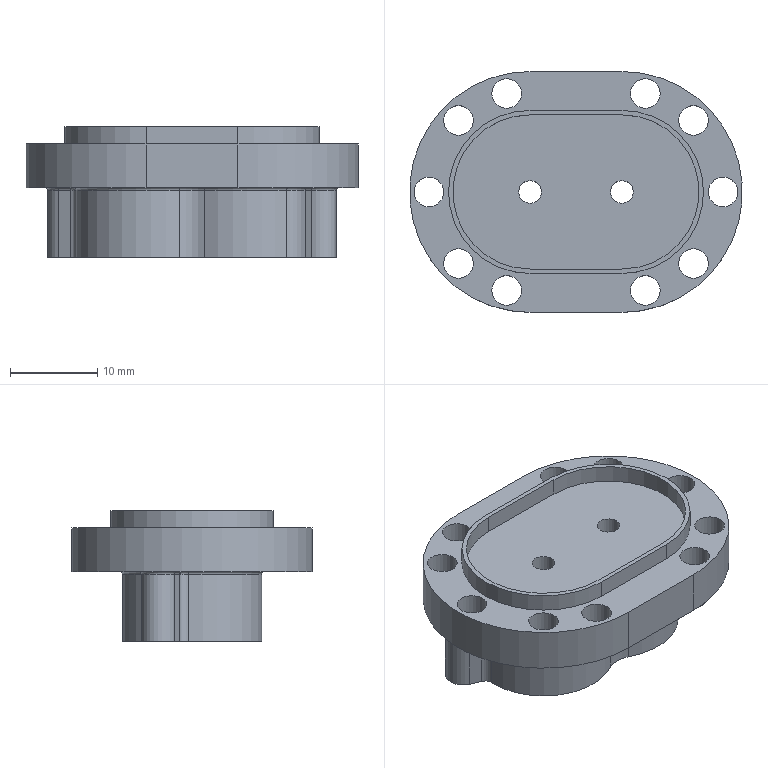Component | NX | END_COVER | 1 solid | 69 faces | volume 5762 mm3 | cylinder 38 | plane 17 | torus 12 | cone 2 | commonest cylinder face diameters 3.4 x10 16 x4 4 x4 0.6 x4 17.668 x2 18.68 x2 6 x2 10 x2